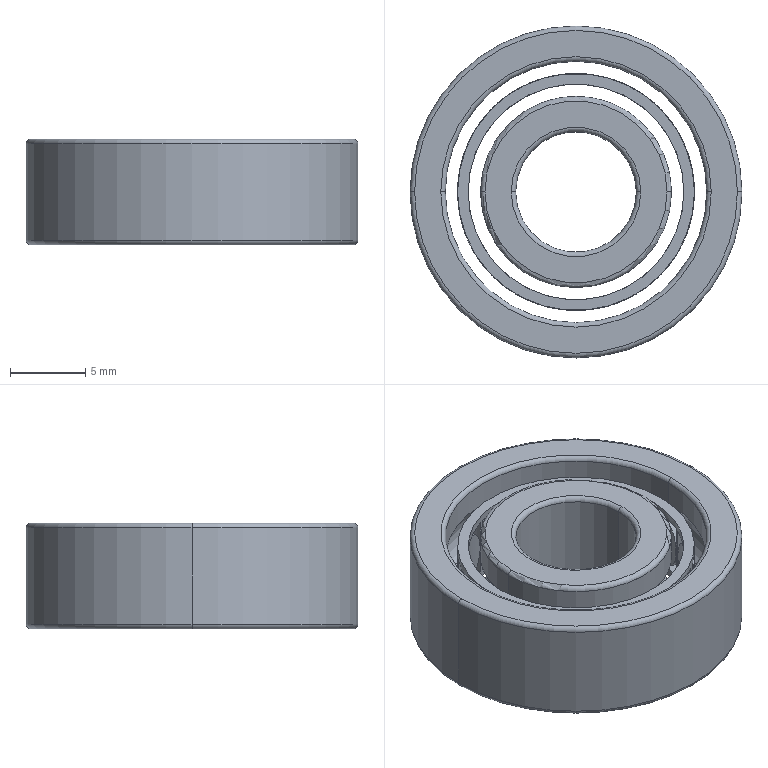Component | SolidWorks | DriveDevice-1_GB_T276-2013[DeepGrooveBallBearing[60000]608]-1 | 14 solids | 136 faces | volume 1512 mm3 | cylinder 64 | plane 28 | sphere 22 | torus 22 | commonest cylinder face diameters 3.95 x24 15.7 x14 14.3 x14 17.333 x4 12.667 x4 22 x2 8 x2 | material AISI 304